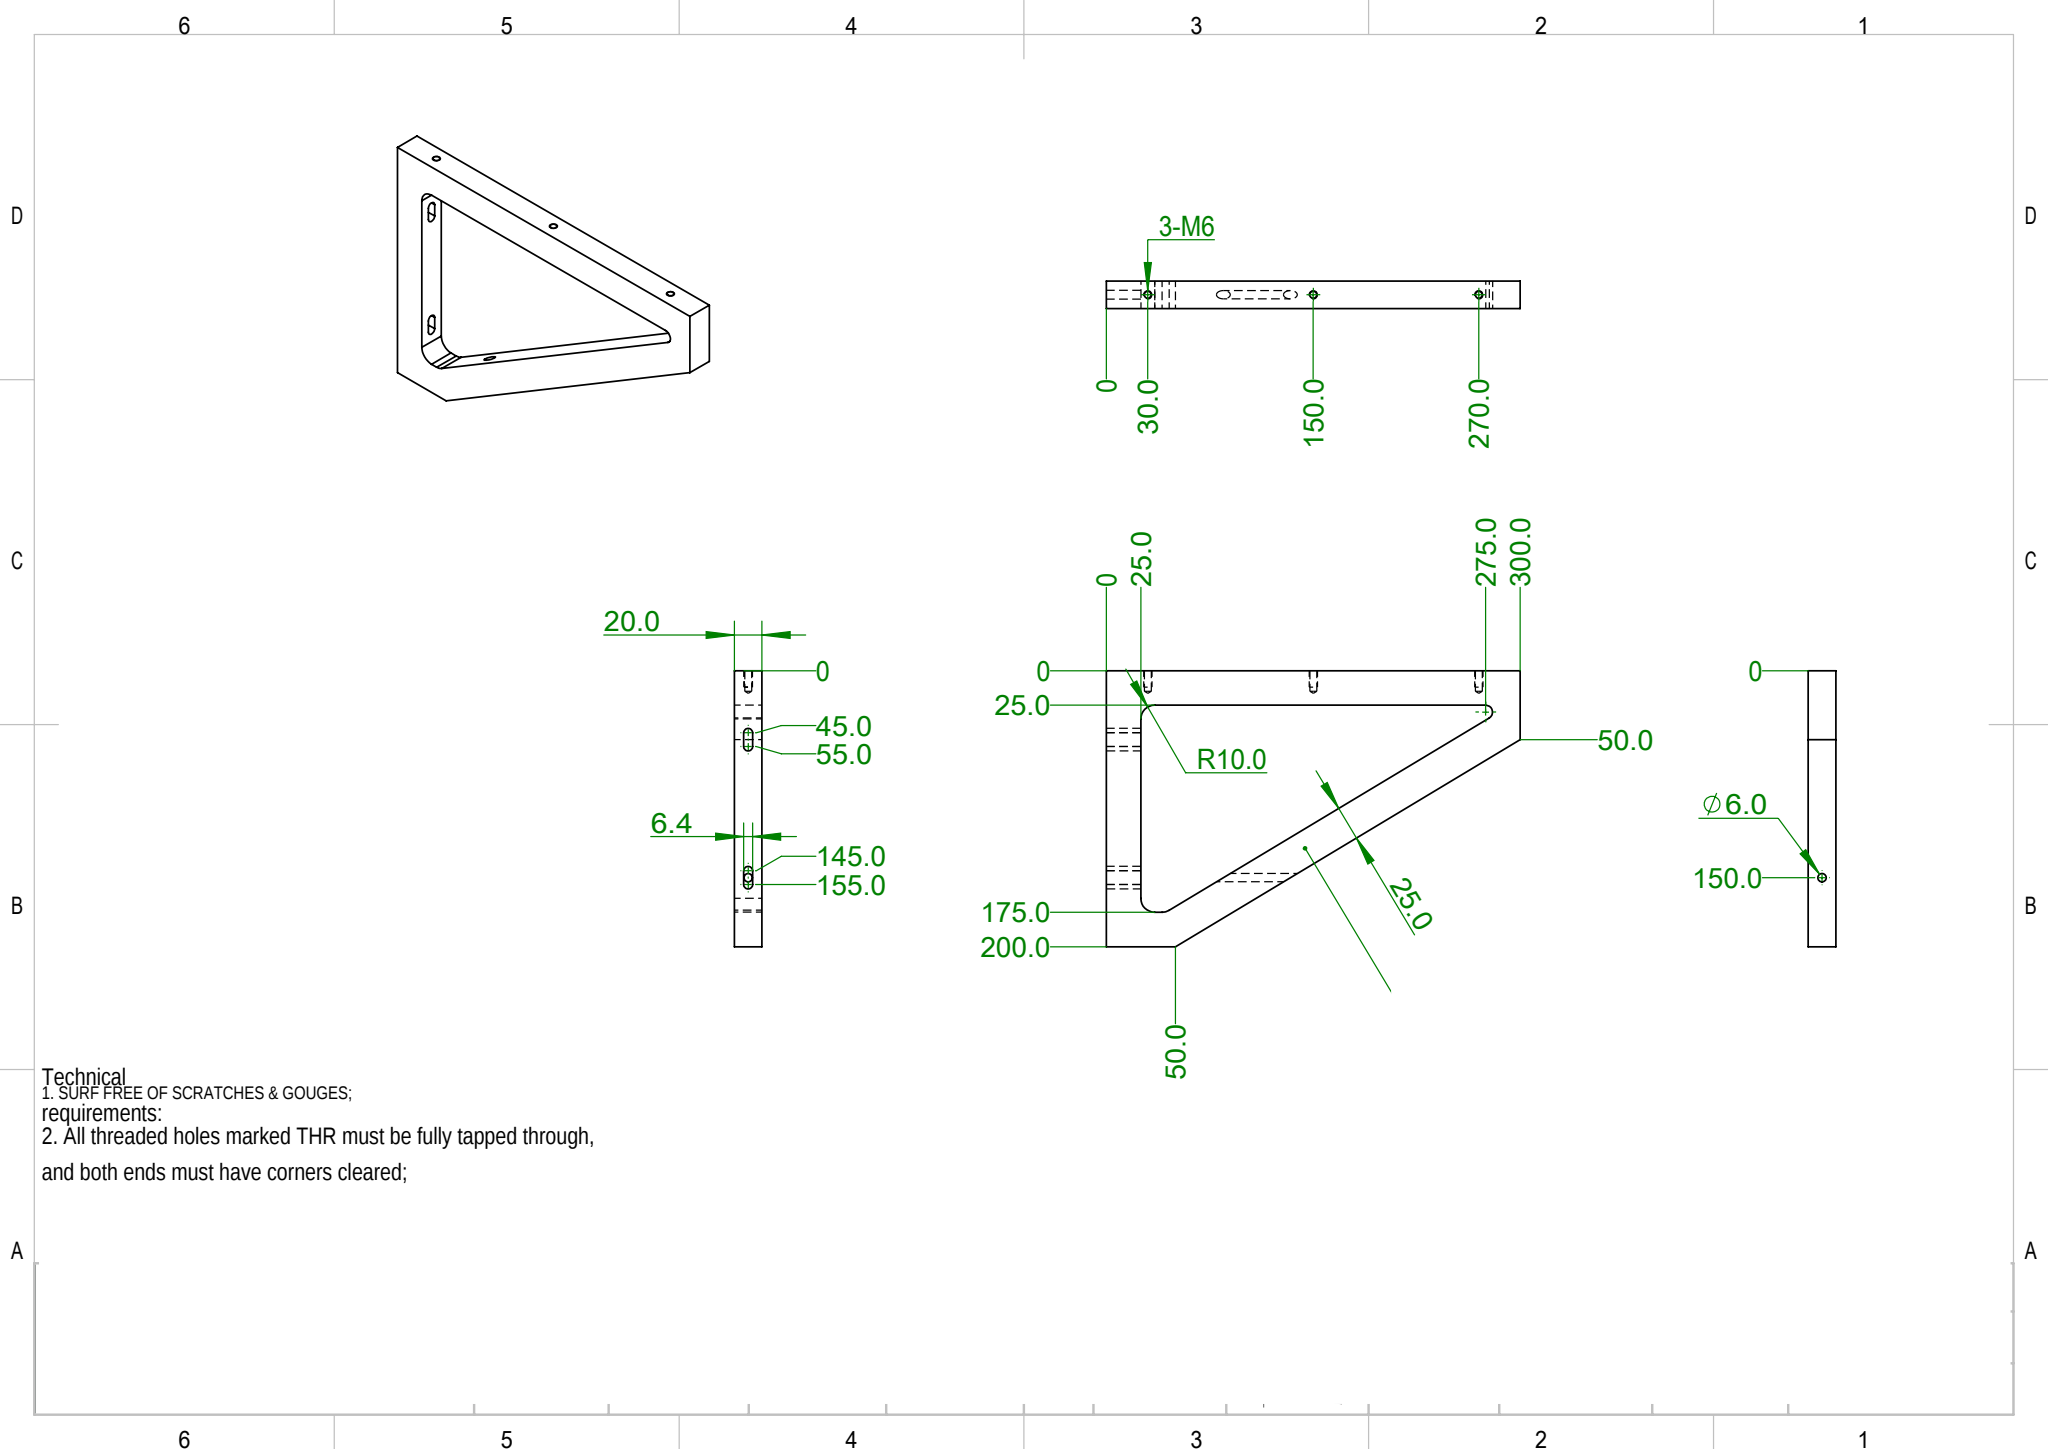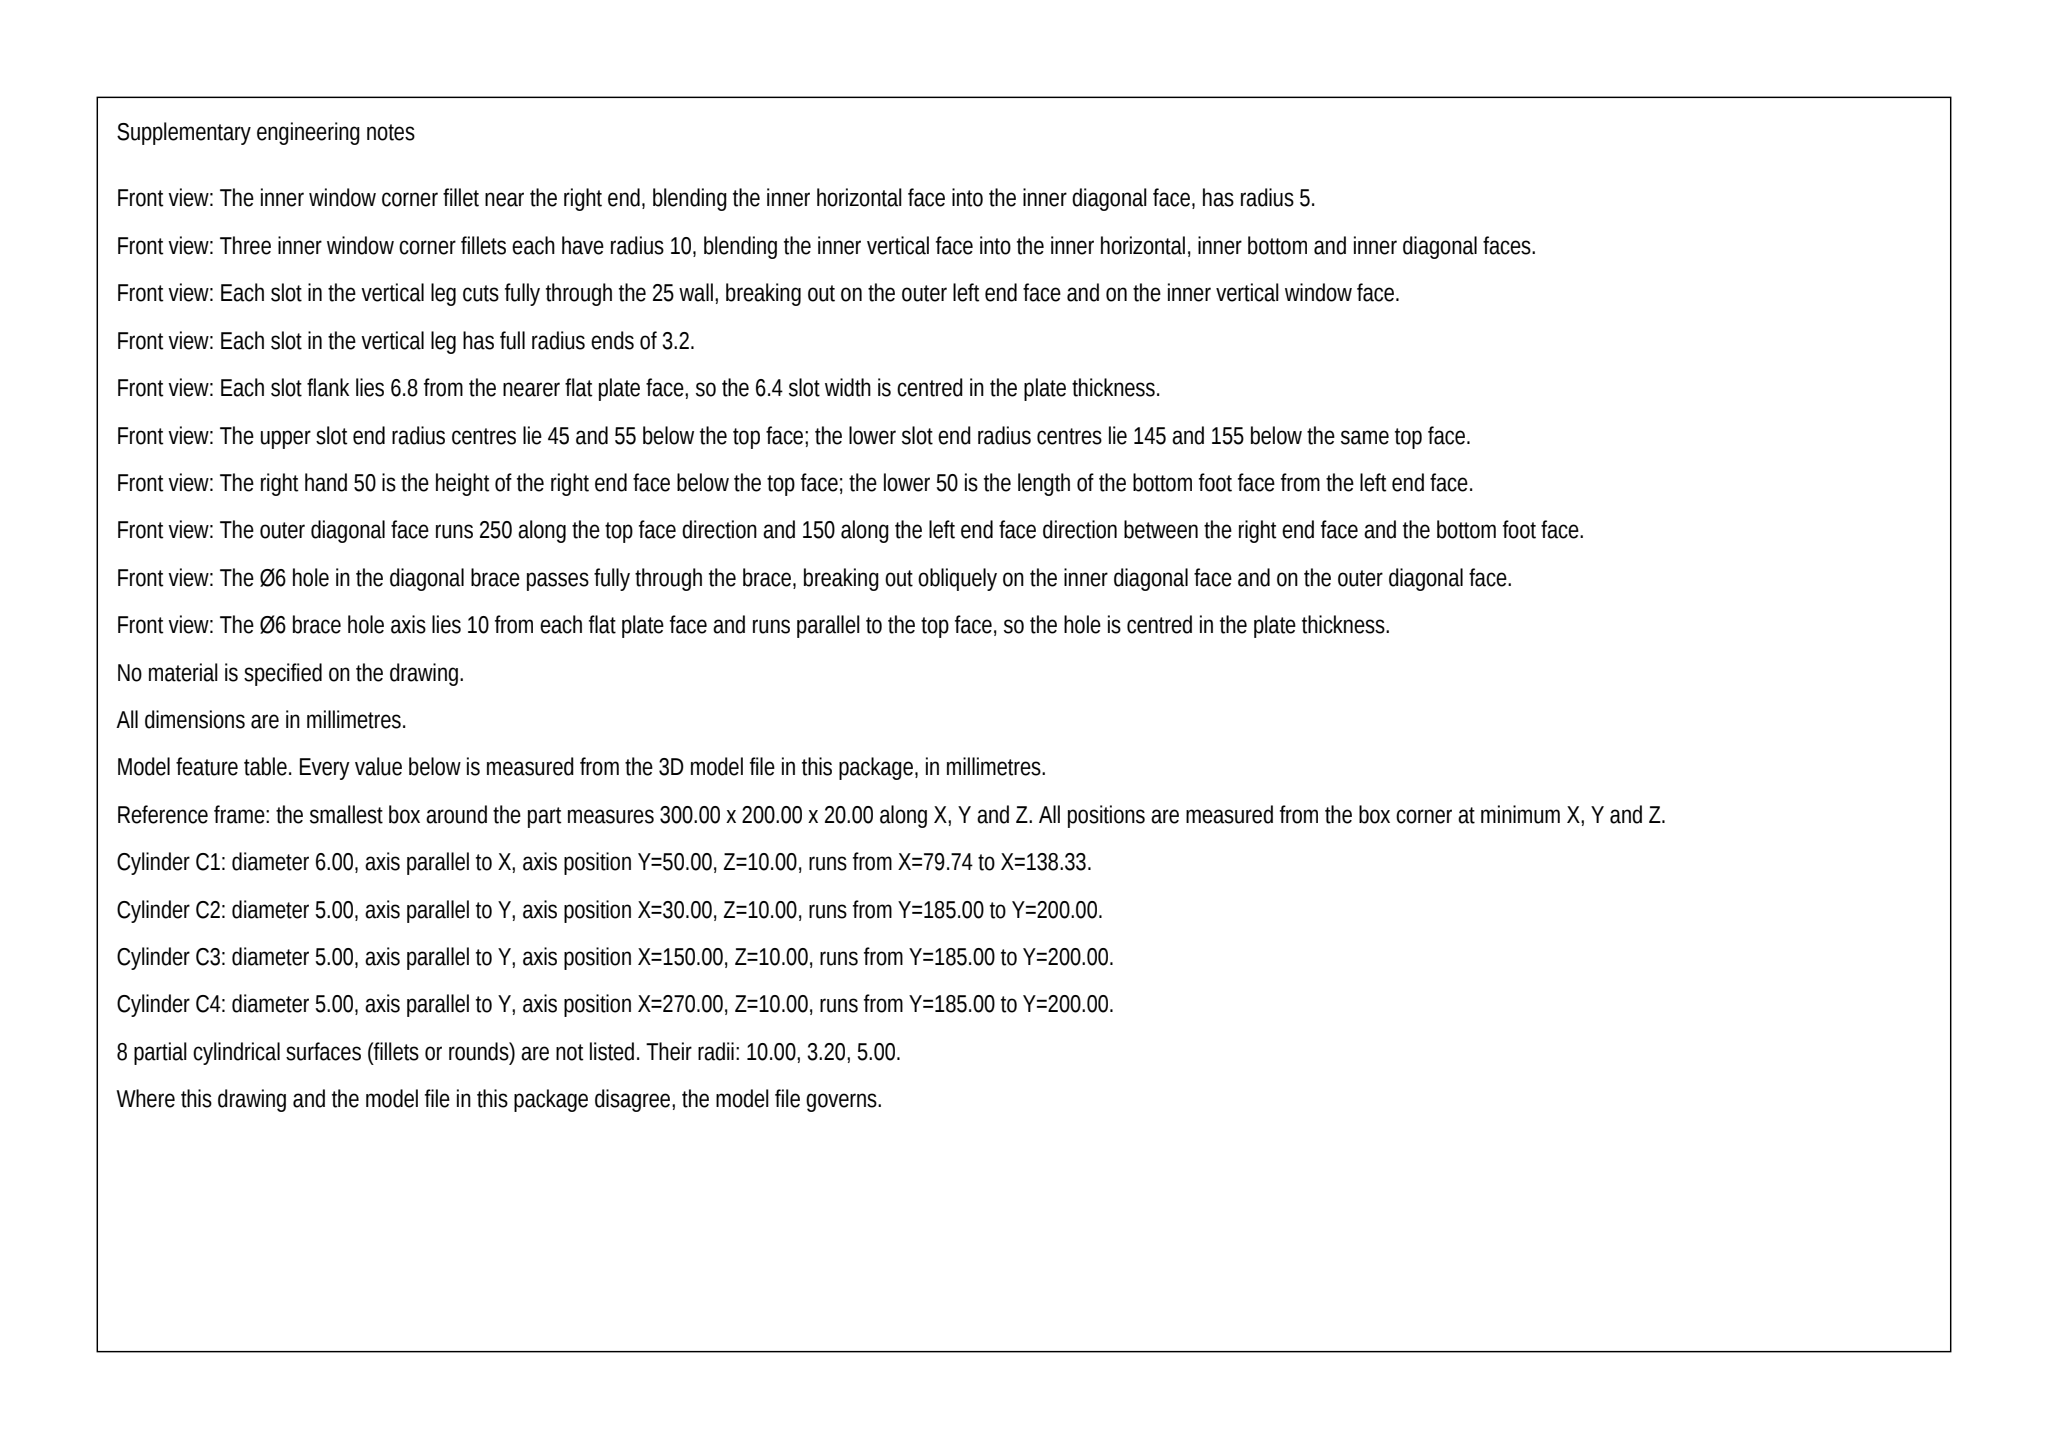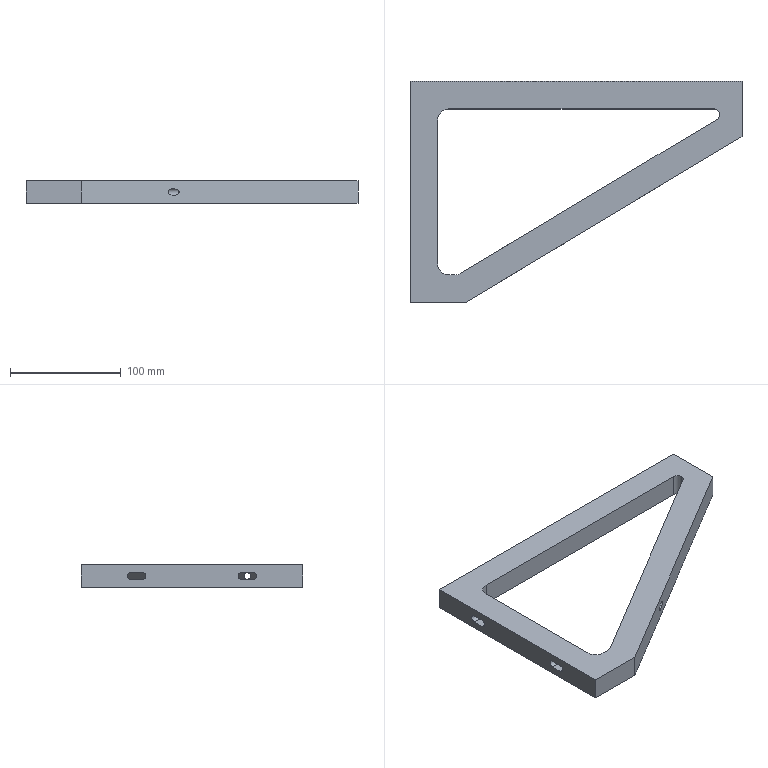Part | SolidWorks | mm | 1 solid | 38 faces | box 300 x 200 x 20 mm | volume 390705 mm3 | cylinder 17 | plane 15 | cone 6 | commonest cylinder face diameters 5 x6 6.4 x4 20 x3 6 x2 10 x2
Drawing notes:
3-M6 DP 15 (BLIND), DRILL Ø5 DP 15, 118° PT | from the solid: Ø5 cylinders, axis Y, length 15 at x=30/150/270, z=10; cone 118° ref dia 5
3-M6 ON CL OF 20 THK LEG: 10 FROM EACH FACE | from the solid: Ø5 Y-axis holes at z=10 in 20 thk plate (z planes 0 and 20)
RH INNER CORNER OF CUTOUT R5 (CTR 275, 30 FROM TOP EDGE) | from the solid: Ø10 Z-axis cylinder at x=275.02, y=170 (=30 from y=200 top edge), len 20
4X 6.4 SLOT IN 25 LEG: CTR 10 FROM EA FACE (Z6.8/13.2) | from the solid: 6.4 dia x-axis cylinders at z=10, planes z=6.8 & 13.2, part thk 20
Ø6.0 THRU: AXIS 10 FROM EA FACE OF 20 THK | from the solid: 6.0 dia x-axis cylinder, pos [y=50, z=10], thk 20 (z planes 0/20)
INNER CUTOUT CORNERS R10 TYP, 3 PLCS | from the solid: Ø20 z-axis cylinders at (35,35), (35,165), (40.31,35) = R10
build123d program:
from build123d import *

# Parameters (mm, degrees)
BOSS_EXTRUDE1_DEPTH   = 10
CUT_EXTRUDE1_DEPTH    = 20
FILLET1_R             = 10
CUT_EXTRUDE2_DEPTH    = 30
SKETCH5_R             = 3
CUT_EXTRUDE4_DEPTH    = 222
M6_TAPPED_HOLE1_D     = 5
M6_TAPPED_HOLE1_DEPTH = 15
M6_TAPPED_HOLE1_TIP   = 1.502


with BuildPart() as part:
    # Sketch1 → Boss-Extrude1 (new, symmetric)
    with BuildSketch(Plane.XY):
        Polygon((-150, 0), (150, 0), (150, -50), (-100, -200), (-150, -200), align=None)
    extrude(amount=BOSS_EXTRUDE1_DEPTH, both=True)

    # Sketch2 → Cut-Extrude1 (cut)
    with BuildSketch(Plane.XY.offset(10)):
        with BuildLine():
            Line((-125, -25), (-125, -175))
            Line((-125, -175), (-106.925, -175))
            Line((-106.925, -175), (127.596, -34.287))
            ThreePointArc((127.596, -34.287), (129.842, -28.665), (125.024, -25))
            Line((125.024, -25), (-125, -25))
        make_face()
    extrude(amount=-CUT_EXTRUDE1_DEPTH, mode=Mode.SUBTRACT)

    # Fillet1
    fillet1_edges = [part.edges().sort_by_distance(p)[0] for p in [
        (-106.925, -175, 0),
        (-125, -175, 0),
        (-125, -25, 0),
    ]]
    fillet(fillet1_edges, radius=FILLET1_R)

    # Sketch3 → Cut-Extrude2 (cut)
    with BuildSketch(Plane.ZY.offset(150)):
        with BuildLine():
            Line((3.2, -45), (3.2, -55))
            ThreePointArc((3.2, -55), (0, -58.2), (-3.2, -55))
            Line((-3.2, -55), (-3.2, -45))
            ThreePointArc((-3.2, -45), (0, -41.8), (3.2, -45))
        make_face()
        with BuildLine():
            Line((-3.2, -155), (-3.2, -145))
            ThreePointArc((-3.2, -145), (0, -141.8), (3.2, -145))
            Line((3.2, -145), (3.2, -155))
            ThreePointArc((3.2, -155), (0, -158.2), (-3.2, -155))
        make_face()
    extrude(amount=-CUT_EXTRUDE2_DEPTH, mode=Mode.SUBTRACT)

    # Sketch5 → Cut-Extrude4 (cut)
    with BuildSketch(Plane(origin=(-125, 0, 0), x_dir=(0, 0, -1), z_dir=(1, 0, 0))):
        with Locations(Location((0, -150, 0), (0, 0, 270))):
            Circle(SKETCH5_R)
    extrude(amount=CUT_EXTRUDE4_DEPTH, mode=Mode.SUBTRACT)

    # M6 Tapped Hole1
    with Locations(Plane(origin=(0, 0, 0), x_dir=(1, 0, 0), z_dir=(0, 1, 0))):
        with Locations((-120, 0), (0, 0), (120, 0)):
            Hole(M6_TAPPED_HOLE1_D / 2, depth=M6_TAPPED_HOLE1_DEPTH)
            with Locations((0, 0, -(M6_TAPPED_HOLE1_DEPTH + M6_TAPPED_HOLE1_TIP / 2))):  # 118° drill point
                Cone(0, M6_TAPPED_HOLE1_D / 2, M6_TAPPED_HOLE1_TIP, mode=Mode.SUBTRACT)


solid = part.part